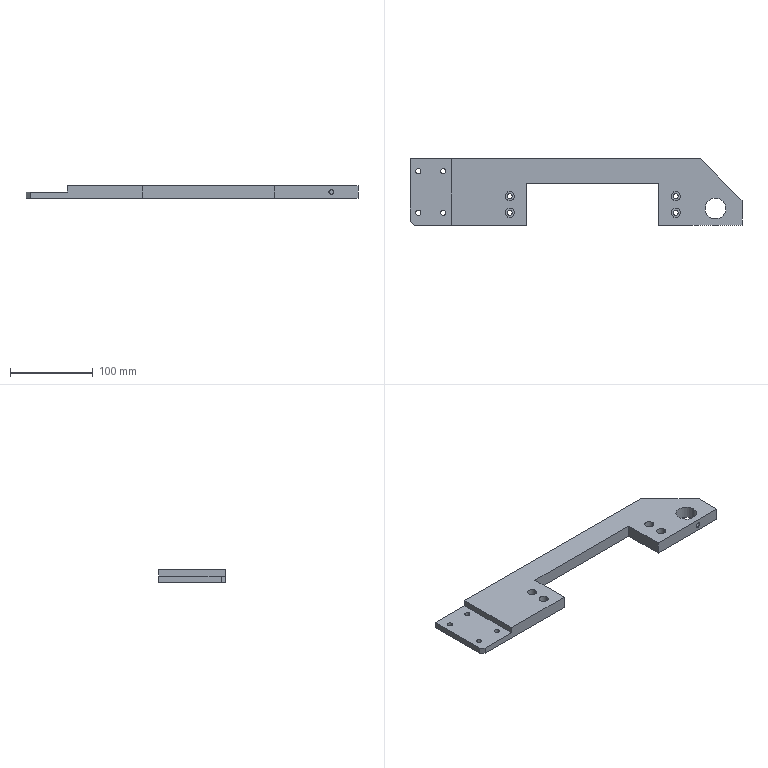Component | SolidWorks | SidePlate(1)-1 | 1 solid | 48 faces | volume 299037 mm3 | cylinder 28 | plane 18 | cone 2 | commonest cylinder face diameters 11 x8 6 x8 6.2 x8 5 x2 25 x2